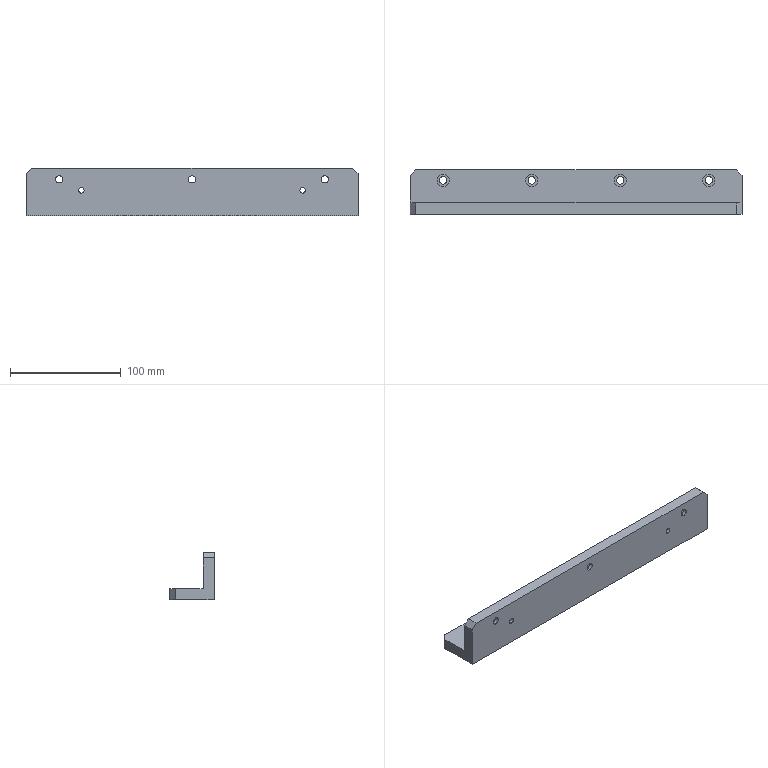Component | SolidWorks | P-SLJ-001-007-2 | 1 solid | 51 faces | box 300 x 40 x 43 mm | volume 212817 mm3 | cylinder 32 | plane 19 | commonest cylinder face diameters 11 x14 6.6 x14 5 x4 | material 45#
build123d program:
from build123d import *

# Parameters (mm, degrees)
EXTRUDE1_DEPTH                                       = 150
CBORE_FOR_M6_HEXAGON_SOCKET_HEAD_CAP_SCR_D           = 6.6
CBORE_FOR_M6_HEXAGON_SOCKET_HEAD_CAP_SCR_CBORE_D     = 11
CBORE_FOR_M6_HEXAGON_SOCKET_HEAD_CAP_SCR_CBORE_DEPTH = 6.8
CBORE_FOR_M6_HEXAGON_SOCKET_HEAD_CAP_2_D             = 6.6
CBORE_FOR_M6_HEXAGON_SOCKET_HEAD_CAP_2_CBORE_D       = 11
CBORE_FOR_M6_HEXAGON_SOCKET_HEAD_CAP_2_CBORE_DEPTH   = 6.8
SIZE_MM_DOWEL_PIN_HOLE1_D                            = 5
CHAMFER1_SIZE                                        = 5


with BuildPart() as part:
    # Sketch1 → Extrude1 (new, symmetric)
    with BuildSketch(Plane(origin=(0, 0, 0), x_dir=(0, 0, -1), z_dir=(1, 0, 0))):
        Polygon((0, 0), (-43, 0), (-43, 10), (-10, 10), (-10, 40), (0, 40), align=None)
    extrude(amount=EXTRUDE1_DEPTH, both=True)

    # CBORE for M6 Hexagon socket head cap scr (through all)
    with Locations(Plane.XY.offset(10)):
        with Locations((-120, 30.5), (-40, 30.5), (40, 30.5), (120, 30.5)):
            CounterBoreHole(CBORE_FOR_M6_HEXAGON_SOCKET_HEAD_CAP_SCR_D / 2, CBORE_FOR_M6_HEXAGON_SOCKET_HEAD_CAP_SCR_CBORE_D / 2, CBORE_FOR_M6_HEXAGON_SOCKET_HEAD_CAP_SCR_CBORE_DEPTH)

    # CBORE for M6 Hexagon socket head cap 2 (through all)
    with Locations(Plane(origin=(0, 10, 0), x_dir=(1, 0, 0), z_dir=(0, 1, 0))):
        with Locations((-120, -33), (0, -33), (120, -33)):
            CounterBoreHole(CBORE_FOR_M6_HEXAGON_SOCKET_HEAD_CAP_2_D / 2, CBORE_FOR_M6_HEXAGON_SOCKET_HEAD_CAP_2_CBORE_D / 2, CBORE_FOR_M6_HEXAGON_SOCKET_HEAD_CAP_2_CBORE_DEPTH)

    # Size mm Dowel Pin Hole1 (through all)
    with Locations(Plane(origin=(0, 10, 0), x_dir=(1, 0, 0), z_dir=(0, 1, 0))):
        with Locations((-100, -23), (100, -23)):
            Hole(SIZE_MM_DOWEL_PIN_HOLE1_D / 2)

    # Chamfer1
    chamfer1_edges = [part.edges().sort_by_distance(p)[0] for p in [
        (150, 5, 43),
        (-150, 5, 43),
        (150, 40, 5),
        (-150, 40, 5),
    ]]
    chamfer(chamfer1_edges, length=CHAMFER1_SIZE)


solid = part.part

# Placed as in the assembly
solid = solid.moved(Location((81.5, -100.5, 1235.634), (0, 0, 0)))